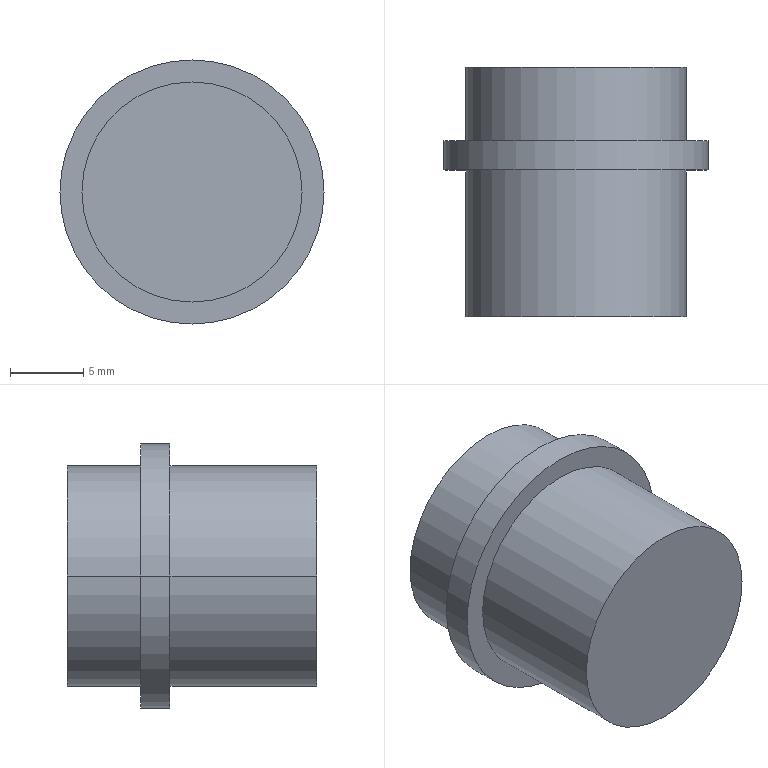Component | SolidWorks | AviationPlug-1 | 1 solid | 24 faces | box 18 x 17 x 18 mm | volume 1920 mm3 | cylinder 15 | plane 9 | commonest cylinder face diameters 2 x7 15 x4 13 x2 18 x2
build123d program:
from build123d import *

# Parameters (mm, degrees)
SKETCH1_R           = 9
BOSS_EXTRUDE1_DEPTH = 2
SKETCH2_R           = 7.5
BOSS_EXTRUDE2_DEPTH = 5
BOSS_EXTRUDE3_START = 10
SKETCH4_R           = 7.5
BOSS_EXTRUDE3_DEPTH = 10
SKETCH3_R           = 1
CUT_EXTRUDE1_DEPTH  = 10
SKETCH5_R           = 6.5
CUT_EXTRUDE2_DEPTH  = 2


with BuildPart() as part:
    # Sketch1 → Boss-Extrude1 (new body)
    with BuildSketch(Plane.XY):
        Circle(SKETCH1_R)
    extrude(amount=BOSS_EXTRUDE1_DEPTH)

    # Sketch2 → Boss-Extrude2 (add)
    with BuildSketch(Plane.XY.offset(2)):
        Circle(SKETCH2_R)
    extrude(amount=BOSS_EXTRUDE2_DEPTH)

    # Sketch4 → Boss-Extrude3 (add)
    with BuildSketch(Plane(origin=(0, 0, 0), x_dir=(-1, 0, 0), z_dir=(0, 0, -1)).offset(BOSS_EXTRUDE3_START)):
        with Locations(Location((0, 0, 0), (0, 0, 180))):
            Circle(SKETCH4_R)
    extrude(amount=-BOSS_EXTRUDE3_DEPTH)

    # Sketch3 → Cut-Extrude1 (cut)
    with BuildSketch(Plane.XY.offset(7)):
        with BuildLine():
            ThreePointArc((-0.997, 6.423), (0, -6.5), (0.997, 6.423))
            ThreePointArc((0.997, 6.423), (0, 5.5), (-0.997, 6.423))
        make_face()
        with Locations((-3.25, 1.876)):
            Circle(SKETCH3_R, mode=Mode.SUBTRACT)
        with Locations((3.25, 1.876)):
            Circle(SKETCH3_R, mode=Mode.SUBTRACT)
        with Locations((0, -3.753)):
            Circle(SKETCH3_R, mode=Mode.SUBTRACT)
    extrude(amount=-CUT_EXTRUDE1_DEPTH, mode=Mode.SUBTRACT)

    # Sketch5 → Cut-Extrude2 (cut)
    with BuildSketch(Plane.XY.offset(7)):
        Circle(SKETCH5_R)
    extrude(amount=-CUT_EXTRUDE2_DEPTH, mode=Mode.SUBTRACT)


solid = part.part

# Placed as in the assembly
solid = solid.moved(Location((1197.686, 1563.312, 2265.983), (-90, 0, 0)))
STEP:
#1=CARTESIAN_POINT('',(46.897,61.43,89.212));
#2=VERTEX_POINT('',#1);
#3=CARTESIAN_POINT('',(47.409,61.43,89.212));
#4=VERTEX_POINT('',#3);
#5=CARTESIAN_POINT('',(47.153,61.43,89.212));
#6=DIRECTION('',(0.,1.,0.));
#7=DIRECTION('',(1.,0.,0.));
#8=AXIS2_PLACEMENT_3D('',#5,#6,#7);
#9=CIRCLE('',#8,0.2559);
#10=EDGE_CURVE('',#2,#4,#9,.T.);
#11=ORIENTED_EDGE('',*,*,#10,.F.);
#12=CARTESIAN_POINT('',(46.897,61.823,89.212));
#13=VERTEX_POINT('',#12);
#14=CARTESIAN_POINT('',(46.897,61.43,89.212));
#15=DIRECTION('',(0.,1.,0.));
#16=VECTOR('',#15,39.37);
#17=LINE('',#14,#16);
#18=EDGE_CURVE('',#2,#13,#17,.T.);
#19=ORIENTED_EDGE('',*,*,#18,.T.);
#20=CARTESIAN_POINT('',(47.409,61.823,89.212));
#21=VERTEX_POINT('',#20);
#22=CARTESIAN_POINT('',(47.153,61.823,89.212));
#23=DIRECTION('',(0.,1.,0.));
#24=DIRECTION('',(1.,0.,0.));
#25=AXIS2_PLACEMENT_3D('',#22,#23,#24);
#26=CIRCLE('',#25,0.2559);
#27=EDGE_CURVE('',#13,#21,#26,.T.);
#28=ORIENTED_EDGE('',*,*,#27,.T.);
#29=CARTESIAN_POINT('',(47.409,61.43,89.212));
#30=DIRECTION('',(0.,1.,0.));
#31=VECTOR('',#30,39.37);
#32=LINE('',#29,#31);
#33=EDGE_CURVE('',#4,#21,#32,.T.);
#34=ORIENTED_EDGE('',*,*,#33,.F.);
#35=EDGE_LOOP('',(#11,#19,#28,#34));
#36=FACE_OUTER_BOUND('',#35,.T.);
#37=CARTESIAN_POINT('',(47.153,61.43,89.212));
#38=DIRECTION('',(0.,1.,0.));
#39=DIRECTION('',(1.,0.,0.));
#40=AXIS2_PLACEMENT_3D('',#37,#38,#39);
#41=CYLINDRICAL_SURFACE('',#40,0.2559);
#42=ADVANCED_FACE('',(#36),#41,.F.);
#43=CARTESIAN_POINT('',(46.858,61.154,89.212));
#44=VERTEX_POINT('',#43);
#45=CARTESIAN_POINT('',(47.448,61.154,89.212));
#46=VERTEX_POINT('',#45);
#47=CARTESIAN_POINT('',(47.153,61.154,89.212));
#48=DIRECTION('',(0.,-1.,-0.));
#49=DIRECTION('',(-1.,0.,0.));
#50=AXIS2_PLACEMENT_3D('',#47,#48,#49);
#51=CIRCLE('',#50,0.2953);
#52=EDGE_CURVE('',#44,#46,#51,.T.);
#53=ORIENTED_EDGE('',*,*,#52,.F.);
#54=CARTESIAN_POINT('',(46.858,61.548,89.212));
#55=VERTEX_POINT('',#54);
#56=CARTESIAN_POINT('',(46.858,61.154,89.212));
#57=DIRECTION('',(0.,1.,0.));
#58=VECTOR('',#57,39.37);
#59=LINE('',#56,#58);
#60=EDGE_CURVE('',#44,#55,#59,.T.);
#61=ORIENTED_EDGE('',*,*,#60,.T.);
#62=CARTESIAN_POINT('',(47.448,61.548,89.212));
#63=VERTEX_POINT('',#62);
#64=CARTESIAN_POINT('',(47.153,61.548,89.212));
#65=DIRECTION('',(0.,-1.,-0.));
#66=DIRECTION('',(1.,0.,0.));
#67=AXIS2_PLACEMENT_3D('',#64,#65,#66);
#68=CIRCLE('',#67,0.2953);
#69=EDGE_CURVE('',#55,#63,#68,.T.);
#70=ORIENTED_EDGE('',*,*,#69,.T.);
#71=CARTESIAN_POINT('',(47.448,61.154,89.212));
#72=DIRECTION('',(0.,1.,0.));
#73=VECTOR('',#72,39.37);
#74=LINE('',#71,#73);
#75=EDGE_CURVE('',#46,#63,#74,.T.);
#76=ORIENTED_EDGE('',*,*,#75,.F.);
#77=EDGE_LOOP('',(#53,#61,#70,#76));
#78=FACE_OUTER_BOUND('',#77,.T.);
#79=CARTESIAN_POINT('',(47.153,61.154,89.212));
#80=DIRECTION('',(0.,1.,0.));
#81=DIRECTION('',(1.,0.,0.));
#82=AXIS2_PLACEMENT_3D('',#79,#80,#81);
#83=CYLINDRICAL_SURFACE('',#82,0.2953);
#84=ADVANCED_FACE('',(#78),#83,.T.);
#85=CARTESIAN_POINT('',(47.448,61.823,89.212));
#86=VERTEX_POINT('',#85);
#87=CARTESIAN_POINT('',(46.858,61.823,89.212));
#88=VERTEX_POINT('',#87);
#89=CARTESIAN_POINT('',(47.153,61.823,89.212));
#90=DIRECTION('',(0.,1.,0.));
#91=DIRECTION('',(1.,0.,0.));
#92=AXIS2_PLACEMENT_3D('',#89,#90,#91);
#93=CIRCLE('',#92,0.2953);
#94=EDGE_CURVE('',#86,#88,#93,.T.);
#95=ORIENTED_EDGE('',*,*,#94,.F.);
#96=CARTESIAN_POINT('',(47.448,61.626,89.212));
#97=VERTEX_POINT('',#96);
#98=CARTESIAN_POINT('',(47.448,61.823,89.212));
#99=DIRECTION('',(0.,-1.,-0.));
#100=VECTOR('',#99,39.37);
#101=LINE('',#98,#100);
#102=EDGE_CURVE('',#86,#97,#101,.T.);
#103=ORIENTED_EDGE('',*,*,#102,.T.);
#104=CARTESIAN_POINT('',(46.858,61.626,89.212));
#105=VERTEX_POINT('',#104);
#106=CARTESIAN_POINT('',(47.153,61.626,89.212));
#107=DIRECTION('',(0.,1.,0.));
#108=DIRECTION('',(1.,0.,0.));
#109=AXIS2_PLACEMENT_3D('',#106,#107,#108);
#110=CIRCLE('',#109,0.2953);
#111=EDGE_CURVE('',#97,#105,#110,.T.);
#112=ORIENTED_EDGE('',*,*,#111,.T.);
#113=CARTESIAN_POINT('',(46.858,61.823,89.212));
#114=DIRECTION('',(0.,-1.,-0.));
#115=VECTOR('',#114,39.37);
#116=LINE('',#113,#115);
#117=EDGE_CURVE('',#88,#105,#116,.T.);
#118=ORIENTED_EDGE('',*,*,#117,.F.);
#119=EDGE_LOOP('',(#95,#103,#112,#118));
#120=FACE_OUTER_BOUND('',#119,.T.);
#121=CARTESIAN_POINT('',(47.153,61.823,89.212));
#122=DIRECTION('',(0.,-1.,-0.));
#123=DIRECTION('',(-1.,0.,0.));
#124=AXIS2_PLACEMENT_3D('',#121,#122,#123);
#125=CYLINDRICAL_SURFACE('',#124,0.2953);
#126=ADVANCED_FACE('',(#120),#125,.T.);
#127=CARTESIAN_POINT('',(47.507,61.626,89.212));
#128=VERTEX_POINT('',#127);
#129=CARTESIAN_POINT('',(46.799,61.626,89.212));
#130=VERTEX_POINT('',#129);
#131=CARTESIAN_POINT('',(47.153,61.626,89.212));
#132=DIRECTION('',(0.,1.,0.));
#133=DIRECTION('',(1.,0.,0.));
#134=AXIS2_PLACEMENT_3D('',#131,#132,#133);
#135=CIRCLE('',#134,0.3543);
#136=EDGE_CURVE('',#128,#130,#135,.T.);
#137=ORIENTED_EDGE('',*,*,#136,.F.);
#138=CARTESIAN_POINT('',(47.507,61.548,89.212));
#139=VERTEX_POINT('',#138);
#140=CARTESIAN_POINT('',(47.507,61.626,89.212));
#141=DIRECTION('',(0.,-1.,-0.));
#142=VECTOR('',#141,39.37);
#143=LINE('',#140,#142);
#144=EDGE_CURVE('',#128,#139,#143,.T.);
#145=ORIENTED_EDGE('',*,*,#144,.T.);
#146=CARTESIAN_POINT('',(46.799,61.548,89.212));
#147=VERTEX_POINT('',#146);
#148=CARTESIAN_POINT('',(47.153,61.548,89.212));
#149=DIRECTION('',(0.,1.,0.));
#150=DIRECTION('',(1.,0.,0.));
#151=AXIS2_PLACEMENT_3D('',#148,#149,#150);
#152=CIRCLE('',#151,0.3543);
#153=EDGE_CURVE('',#139,#147,#152,.T.);
#154=ORIENTED_EDGE('',*,*,#153,.T.);
#155=CARTESIAN_POINT('',(46.799,61.626,89.212));
#156=DIRECTION('',(0.,-1.,-0.));
#157=VECTOR('',#156,39.37);
#158=LINE('',#155,#157);
#159=EDGE_CURVE('',#130,#147,#158,.T.);
#160=ORIENTED_EDGE('',*,*,#159,.F.);
#161=EDGE_LOOP('',(#137,#145,#154,#160));
#162=FACE_OUTER_BOUND('',#161,.T.);
#163=CARTESIAN_POINT('',(47.153,61.626,89.212));
#164=DIRECTION('',(0.,-1.,-0.));
#165=DIRECTION('',(-1.,0.,0.));
#166=AXIS2_PLACEMENT_3D('',#163,#164,#165);
#167=CYLINDRICAL_SURFACE('',#166,0.3543);
#168=ADVANCED_FACE('',(#162),#167,.T.);
#169=CARTESIAN_POINT('',(47.192,61.43,89.36));
#170=VERTEX_POINT('',#169);
#171=CARTESIAN_POINT('',(47.114,61.43,89.36));
#172=VERTEX_POINT('',#171);
#173=CARTESIAN_POINT('',(47.153,61.43,89.36));
#174=DIRECTION('',(0.,1.,0.));
#175=DIRECTION('',(1.,0.,0.));
#176=AXIS2_PLACEMENT_3D('',#173,#174,#175);
#177=CIRCLE('',#176,0.03937);
#178=EDGE_CURVE('',#170,#172,#177,.T.);
#179=ORIENTED_EDGE('',*,*,#178,.T.);
#180=CARTESIAN_POINT('',(47.114,61.745,89.36));
#181=VERTEX_POINT('',#180);
#182=CARTESIAN_POINT('',(47.114,61.43,89.36));
#183=DIRECTION('',(0.,1.,0.));
#184=VECTOR('',#183,39.37);
#185=LINE('',#182,#184);
#186=EDGE_CURVE('',#172,#181,#185,.T.);
#187=ORIENTED_EDGE('',*,*,#186,.T.);
#188=CARTESIAN_POINT('',(47.192,61.745,89.36));
#189=VERTEX_POINT('',#188);
#190=CARTESIAN_POINT('',(47.153,61.745,89.36));
#191=DIRECTION('',(0.,-1.,-0.));
#192=DIRECTION('',(1.,0.,0.));
#193=AXIS2_PLACEMENT_3D('',#190,#191,#192);
#194=CIRCLE('',#193,0.03937);
#195=EDGE_CURVE('',#181,#189,#194,.T.);
#196=ORIENTED_EDGE('',*,*,#195,.T.);
#197=CARTESIAN_POINT('',(47.192,61.43,89.36));
#198=DIRECTION('',(0.,1.,0.));
#199=VECTOR('',#198,39.37);
#200=LINE('',#197,#199);
#201=EDGE_CURVE('',#170,#189,#200,.T.);
#202=ORIENTED_EDGE('',*,*,#201,.F.);
#203=EDGE_LOOP('',(#179,#187,#196,#202));
#204=FACE_OUTER_BOUND('',#203,.T.);
#205=CARTESIAN_POINT('',(47.153,61.43,89.36));
#206=DIRECTION('',(0.,1.,0.));
#207=DIRECTION('',(1.,0.,0.));
#208=AXIS2_PLACEMENT_3D('',#205,#206,#207);
#209=CYLINDRICAL_SURFACE('',#208,0.03937);
#210=ADVANCED_FACE('',(#204),#209,.T.);
#211=CARTESIAN_POINT('',(47.32,61.43,89.138));
#212=VERTEX_POINT('',#211);
#213=CARTESIAN_POINT('',(47.242,61.43,89.138));
#214=VERTEX_POINT('',#213);
#215=CARTESIAN_POINT('',(47.281,61.43,89.138));
#216=DIRECTION('',(0.,1.,0.));
#217=DIRECTION('',(1.,0.,0.));
#218=AXIS2_PLACEMENT_3D('',#215,#216,#217);
#219=CIRCLE('',#218,0.03937);
#220=EDGE_CURVE('',#212,#214,#219,.T.);
#221=ORIENTED_EDGE('',*,*,#220,.T.);
#222=CARTESIAN_POINT('',(47.242,61.745,89.138));
#223=VERTEX_POINT('',#222);
#224=CARTESIAN_POINT('',(47.242,61.43,89.138));
#225=DIRECTION('',(0.,1.,0.));
#226=VECTOR('',#225,39.37);
#227=LINE('',#224,#226);
#228=EDGE_CURVE('',#214,#223,#227,.T.);
#229=ORIENTED_EDGE('',*,*,#228,.T.);
#230=CARTESIAN_POINT('',(47.32,61.745,89.138));
#231=VERTEX_POINT('',#230);
#232=CARTESIAN_POINT('',(47.281,61.745,89.138));
#233=DIRECTION('',(0.,-1.,-0.));
#234=DIRECTION('',(1.,0.,0.));
#235=AXIS2_PLACEMENT_3D('',#232,#233,#234);
#236=CIRCLE('',#235,0.03937);
#237=EDGE_CURVE('',#223,#231,#236,.T.);
#238=ORIENTED_EDGE('',*,*,#237,.T.);
#239=CARTESIAN_POINT('',(47.32,61.43,89.138));
#240=DIRECTION('',(0.,1.,0.));
#241=VECTOR('',#240,39.37);
#242=LINE('',#239,#241);
#243=EDGE_CURVE('',#212,#231,#242,.T.);
#244=ORIENTED_EDGE('',*,*,#243,.F.);
#245=EDGE_LOOP('',(#221,#229,#238,#244));
#246=FACE_OUTER_BOUND('',#245,.T.);
#247=CARTESIAN_POINT('',(47.281,61.43,89.138));
#248=DIRECTION('',(0.,1.,0.));
#249=DIRECTION('',(1.,0.,0.));
#250=AXIS2_PLACEMENT_3D('',#247,#248,#249);
#251=CYLINDRICAL_SURFACE('',#250,0.03937);
#252=ADVANCED_FACE('',(#246),#251,.T.);
#253=CARTESIAN_POINT('',(47.064,61.43,89.138));
#254=VERTEX_POINT('',#253);
#255=CARTESIAN_POINT('',(46.986,61.43,89.138));
#256=VERTEX_POINT('',#255);
#257=CARTESIAN_POINT('',(47.025,61.43,89.138));
#258=DIRECTION('',(0.,1.,0.));
#259=DIRECTION('',(1.,0.,0.));
#260=AXIS2_PLACEMENT_3D('',#257,#258,#259);
#261=CIRCLE('',#260,0.03937);
#262=EDGE_CURVE('',#254,#256,#261,.T.);
#263=ORIENTED_EDGE('',*,*,#262,.T.);
#264=CARTESIAN_POINT('',(46.986,61.745,89.138));
#265=VERTEX_POINT('',#264);
#266=CARTESIAN_POINT('',(46.986,61.43,89.138));
#267=DIRECTION('',(0.,1.,0.));
#268=VECTOR('',#267,39.37);
#269=LINE('',#266,#268);
#270=EDGE_CURVE('',#256,#265,#269,.T.);
#271=ORIENTED_EDGE('',*,*,#270,.T.);
#272=CARTESIAN_POINT('',(47.064,61.745,89.138));
#273=VERTEX_POINT('',#272);
#274=CARTESIAN_POINT('',(47.025,61.745,89.138));
#275=DIRECTION('',(0.,-1.,-0.));
#276=DIRECTION('',(1.,0.,0.));
#277=AXIS2_PLACEMENT_3D('',#274,#275,#276);
#278=CIRCLE('',#277,0.03937);
#279=EDGE_CURVE('',#265,#273,#278,.T.);
#280=ORIENTED_EDGE('',*,*,#279,.T.);
#281=CARTESIAN_POINT('',(47.064,61.43,89.138));
#282=DIRECTION('',(0.,1.,0.));
#283=VECTOR('',#282,39.37);
#284=LINE('',#281,#283);
#285=EDGE_CURVE('',#254,#273,#284,.T.);
#286=ORIENTED_EDGE('',*,*,#285,.F.);
#287=EDGE_LOOP('',(#263,#271,#280,#286));
#288=FACE_OUTER_BOUND('',#287,.T.);
#289=CARTESIAN_POINT('',(47.025,61.43,89.138));
#290=DIRECTION('',(0.,1.,0.));
#291=DIRECTION('',(1.,0.,0.));
#292=AXIS2_PLACEMENT_3D('',#289,#290,#291);
#293=CYLINDRICAL_SURFACE('',#292,0.03937);
#294=ADVANCED_FACE('',(#288),#293,.T.);
#295=CARTESIAN_POINT('',(47.114,61.745,88.959));
#296=VERTEX_POINT('',#295);
#297=CARTESIAN_POINT('',(47.192,61.745,88.959));
#298=VERTEX_POINT('',#297);
#299=CARTESIAN_POINT('',(47.153,61.745,88.956));
#300=DIRECTION('',(0.,1.,0.));
#301=DIRECTION('',(1.,0.,0.));
#302=AXIS2_PLACEMENT_3D('',#299,#300,#301);
#303=CIRCLE('',#302,0.03937);
#304=EDGE_CURVE('',#296,#298,#303,.T.);
#305=ORIENTED_EDGE('',*,*,#304,.F.);
#306=CARTESIAN_POINT('',(47.114,61.43,88.959));
#307=VERTEX_POINT('',#306);
#308=CARTESIAN_POINT('',(47.114,61.43,88.959));
#309=DIRECTION('',(0.,1.,0.));
#310=VECTOR('',#309,39.37);
#311=LINE('',#308,#310);
#312=EDGE_CURVE('',#307,#296,#311,.T.);
#313=ORIENTED_EDGE('',*,*,#312,.F.);
#314=CARTESIAN_POINT('',(47.192,61.43,88.959));
#315=VERTEX_POINT('',#314);
#316=CARTESIAN_POINT('',(47.153,61.43,88.956));
#317=DIRECTION('',(0.,-1.,-0.));
#318=DIRECTION('',(1.,0.,0.));
#319=AXIS2_PLACEMENT_3D('',#316,#317,#318);
#320=CIRCLE('',#319,0.03937);
#321=EDGE_CURVE('',#315,#307,#320,.T.);
#322=ORIENTED_EDGE('',*,*,#321,.F.);
#323=CARTESIAN_POINT('',(47.192,61.43,88.959));
#324=DIRECTION('',(0.,1.,0.));
#325=VECTOR('',#324,39.37);
#326=LINE('',#323,#325);
#327=EDGE_CURVE('',#315,#298,#326,.T.);
#328=ORIENTED_EDGE('',*,*,#327,.T.);
#329=EDGE_LOOP('',(#305,#313,#322,#328));
#330=FACE_OUTER_BOUND('',#329,.T.);
#331=CARTESIAN_POINT('',(47.153,61.43,88.956));
#332=DIRECTION('',(0.,1.,0.));
#333=DIRECTION('',(1.,0.,0.));
#334=AXIS2_PLACEMENT_3D('',#331,#332,#333);
#335=CYLINDRICAL_SURFACE('',#334,0.03937);
#336=ADVANCED_FACE('',(#330),#335,.T.);
#337=ORIENTED_EDGE('',*,*,#270,.F.);
#338=CARTESIAN_POINT('',(47.025,61.43,89.138));
#339=DIRECTION('',(0.,1.,0.));
#340=DIRECTION('',(1.,0.,0.));
#341=AXIS2_PLACEMENT_3D('',#338,#339,#340);
#342=CIRCLE('',#341,0.03937);
#343=EDGE_CURVE('',#256,#254,#342,.T.);
#344=ORIENTED_EDGE('',*,*,#343,.T.);
#345=ORIENTED_EDGE('',*,*,#285,.T.);
#346=CARTESIAN_POINT('',(47.025,61.745,89.138));
#347=DIRECTION('',(0.,-1.,-0.));
#348=DIRECTION('',(1.,0.,0.));
#349=AXIS2_PLACEMENT_3D('',#346,#347,#348);
#350=CIRCLE('',#349,0.03937);
#351=EDGE_CURVE('',#273,#265,#350,.T.);
#352=ORIENTED_EDGE('',*,*,#351,.T.);
#353=EDGE_LOOP('',(#337,#344,#345,#352));
#354=FACE_OUTER_BOUND('',#353,.T.);
#355=CARTESIAN_POINT('',(47.025,61.43,89.138));
#356=DIRECTION('',(0.,1.,0.));
#357=DIRECTION('',(1.,0.,0.));
#358=AXIS2_PLACEMENT_3D('',#355,#356,#357);
#359=CYLINDRICAL_SURFACE('',#358,0.03937);
#360=ADVANCED_FACE('',(#354),#359,.T.);
#361=ORIENTED_EDGE('',*,*,#228,.F.);
#362=CARTESIAN_POINT('',(47.281,61.43,89.138));
#363=DIRECTION('',(0.,1.,0.));
#364=DIRECTION('',(1.,0.,0.));
#365=AXIS2_PLACEMENT_3D('',#362,#363,#364);
#366=CIRCLE('',#365,0.03937);
#367=EDGE_CURVE('',#214,#212,#366,.T.);
#368=ORIENTED_EDGE('',*,*,#367,.T.);
#369=ORIENTED_EDGE('',*,*,#243,.T.);
#370=CARTESIAN_POINT('',(47.281,61.745,89.138));
#371=DIRECTION('',(0.,-1.,-0.));
#372=DIRECTION('',(1.,0.,0.));
#373=AXIS2_PLACEMENT_3D('',#370,#371,#372);
#374=CIRCLE('',#373,0.03937);
#375=EDGE_CURVE('',#231,#223,#374,.T.);
#376=ORIENTED_EDGE('',*,*,#375,.T.);
#377=EDGE_LOOP('',(#361,#368,#369,#376));
#378=FACE_OUTER_BOUND('',#377,.T.);
#379=CARTESIAN_POINT('',(47.281,61.43,89.138));
#380=DIRECTION('',(0.,1.,0.));
#381=DIRECTION('',(1.,0.,0.));
#382=AXIS2_PLACEMENT_3D('',#379,#380,#381);
#383=CYLINDRICAL_SURFACE('',#382,0.03937);
#384=ADVANCED_FACE('',(#378),#383,.T.);
#385=ORIENTED_EDGE('',*,*,#186,.F.);
#386=CARTESIAN_POINT('',(47.153,61.43,89.36));
#387=DIRECTION('',(0.,1.,0.));
#388=DIRECTION('',(1.,0.,0.));
#389=AXIS2_PLACEMENT_3D('',#386,#387,#388);
#390=CIRCLE('',#389,0.03937);
#391=EDGE_CURVE('',#172,#170,#390,.T.);
#392=ORIENTED_EDGE('',*,*,#391,.T.);
#393=ORIENTED_EDGE('',*,*,#201,.T.);
#394=CARTESIAN_POINT('',(47.153,61.745,89.36));
#395=DIRECTION('',(0.,-1.,-0.));
#396=DIRECTION('',(1.,0.,0.));
#397=AXIS2_PLACEMENT_3D('',#394,#395,#396);
#398=CIRCLE('',#397,0.03937);
#399=EDGE_CURVE('',#189,#181,#398,.T.);
#400=ORIENTED_EDGE('',*,*,#399,.T.);
#401=EDGE_LOOP('',(#385,#392,#393,#400));
#402=FACE_OUTER_BOUND('',#401,.T.);
#403=CARTESIAN_POINT('',(47.153,61.43,89.36));
#404=DIRECTION('',(0.,1.,0.));
#405=DIRECTION('',(1.,0.,0.));
#406=AXIS2_PLACEMENT_3D('',#403,#404,#405);
#407=CYLINDRICAL_SURFACE('',#406,0.03937);
#408=ADVANCED_FACE('',(#402),#407,.T.);
#409=ORIENTED_EDGE('',*,*,#144,.F.);
#410=CARTESIAN_POINT('',(47.153,61.626,89.212));
#411=DIRECTION('',(0.,1.,0.));
#412=DIRECTION('',(1.,0.,0.));
#413=AXIS2_PLACEMENT_3D('',#410,#411,#412);
#414=CIRCLE('',#413,0.3543);
#415=EDGE_CURVE('',#130,#128,#414,.T.);
#416=ORIENTED_EDGE('',*,*,#415,.F.);
#417=ORIENTED_EDGE('',*,*,#159,.T.);
#418=CARTESIAN_POINT('',(47.153,61.548,89.212));
#419=DIRECTION('',(0.,1.,0.));
#420=DIRECTION('',(1.,0.,0.));
#421=AXIS2_PLACEMENT_3D('',#418,#419,#420);
#422=CIRCLE('',#421,0.3543);
#423=EDGE_CURVE('',#147,#139,#422,.T.);
#424=ORIENTED_EDGE('',*,*,#423,.T.);
#425=EDGE_LOOP('',(#409,#416,#417,#424));
#426=FACE_OUTER_BOUND('',#425,.T.);
#427=CARTESIAN_POINT('',(47.153,61.626,89.212));
#428=DIRECTION('',(0.,-1.,-0.));
#429=DIRECTION('',(-1.,0.,0.));
#430=AXIS2_PLACEMENT_3D('',#427,#428,#429);
#431=CYLINDRICAL_SURFACE('',#430,0.3543);
#432=ADVANCED_FACE('',(#426),#431,.T.);
#433=CARTESIAN_POINT('',(47.153,61.626,89.212));
#434=DIRECTION('',(0.,1.,0.));
#435=DIRECTION('',(1.,0.,0.));
#436=AXIS2_PLACEMENT_3D('',#433,#434,#435);
#437=CIRCLE('',#436,0.2953);
#438=EDGE_CURVE('',#105,#97,#437,.T.);
#439=ORIENTED_EDGE('',*,*,#438,.F.);
#440=ORIENTED_EDGE('',*,*,#111,.F.);
#441=EDGE_LOOP('',(#439,#440));
#442=FACE_BOUND('',#441,.T.);
#443=ORIENTED_EDGE('',*,*,#415,.T.);
#444=ORIENTED_EDGE('',*,*,#136,.T.);
#445=EDGE_LOOP('',(#443,#444));
#446=FACE_OUTER_BOUND('',#445,.T.);
#447=CARTESIAN_POINT('',(47.153,61.626,89.212));
#448=DIRECTION('',(0.,1.,0.));
#449=DIRECTION('',(1.,0.,0.));
#450=AXIS2_PLACEMENT_3D('',#447,#448,#449);
#451=PLANE('',#450);
#452=ADVANCED_FACE('',(#442,#446),#451,.T.);
#453=CARTESIAN_POINT('',(47.153,61.548,89.212));
#454=DIRECTION('',(0.,-1.,-0.));
#455=DIRECTION('',(1.,0.,0.));
#456=AXIS2_PLACEMENT_3D('',#453,#454,#455);
#457=CIRCLE('',#456,0.2953);
#458=EDGE_CURVE('',#63,#55,#457,.T.);
#459=ORIENTED_EDGE('',*,*,#458,.F.);
#460=ORIENTED_EDGE('',*,*,#69,.F.);
#461=EDGE_LOOP('',(#459,#460));
#462=FACE_BOUND('',#461,.T.);
#463=ORIENTED_EDGE('',*,*,#423,.F.);
#464=ORIENTED_EDGE('',*,*,#153,.F.);
#465=EDGE_LOOP('',(#463,#464));
#466=FACE_OUTER_BOUND('',#465,.T.);
#467=CARTESIAN_POINT('',(47.153,61.548,89.212));
#468=DIRECTION('',(0.,1.,0.));
#469=DIRECTION('',(1.,0.,0.));
#470=AXIS2_PLACEMENT_3D('',#467,#468,#469);
#471=PLANE('',#470);
#472=ADVANCED_FACE('',(#462,#466),#471,.F.);
#473=ORIENTED_EDGE('',*,*,#102,.F.);
#474=CARTESIAN_POINT('',(47.153,61.823,89.212));
#475=DIRECTION('',(0.,1.,0.));
#476=DIRECTION('',(1.,0.,0.));
#477=AXIS2_PLACEMENT_3D('',#474,#475,#476);
#478=CIRCLE('',#477,0.2953);
#479=EDGE_CURVE('',#88,#86,#478,.T.);
#480=ORIENTED_EDGE('',*,*,#479,.F.);
#481=ORIENTED_EDGE('',*,*,#117,.T.);
#482=ORIENTED_EDGE('',*,*,#438,.T.);
#483=EDGE_LOOP('',(#473,#480,#481,#482));
#484=FACE_OUTER_BOUND('',#483,.T.);
#485=CARTESIAN_POINT('',(47.153,61.823,89.212));
#486=DIRECTION('',(0.,-1.,-0.));
#487=DIRECTION('',(-1.,0.,0.));
#488=AXIS2_PLACEMENT_3D('',#485,#486,#487);
#489=CYLINDRICAL_SURFACE('',#488,0.2953);
#490=ADVANCED_FACE('',(#484),#489,.T.);
#491=CARTESIAN_POINT('',(47.153,61.823,89.212));
#492=DIRECTION('',(0.,1.,0.));
#493=DIRECTION('',(1.,0.,0.));
#494=AXIS2_PLACEMENT_3D('',#491,#492,#493);
#495=CIRCLE('',#494,0.2559);
#496=EDGE_CURVE('',#21,#13,#495,.T.);
#497=ORIENTED_EDGE('',*,*,#496,.F.);
#498=ORIENTED_EDGE('',*,*,#27,.F.);
#499=EDGE_LOOP('',(#497,#498));
#500=FACE_BOUND('',#499,.T.);
#501=ORIENTED_EDGE('',*,*,#479,.T.);
#502=ORIENTED_EDGE('',*,*,#94,.T.);
#503=EDGE_LOOP('',(#501,#502));
#504=FACE_OUTER_BOUND('',#503,.T.);
#505=CARTESIAN_POINT('',(47.153,61.823,89.212));
#506=DIRECTION('',(0.,1.,0.));
#507=DIRECTION('',(1.,0.,0.));
#508=AXIS2_PLACEMENT_3D('',#505,#506,#507);
#509=PLANE('',#508);
#510=ADVANCED_FACE('',(#500,#504),#509,.T.);
#511=ORIENTED_EDGE('',*,*,#60,.F.);
#512=CARTESIAN_POINT('',(47.153,61.154,89.212));
#513=DIRECTION('',(0.,-1.,-0.));
#514=DIRECTION('',(-1.,0.,0.));
#515=AXIS2_PLACEMENT_3D('',#512,#513,#514);
#516=CIRCLE('',#515,0.2953);
#517=EDGE_CURVE('',#46,#44,#516,.T.);
#518=ORIENTED_EDGE('',*,*,#517,.F.);
#519=ORIENTED_EDGE('',*,*,#75,.T.);
#520=ORIENTED_EDGE('',*,*,#458,.T.);
#521=EDGE_LOOP('',(#511,#518,#519,#520));
#522=FACE_OUTER_BOUND('',#521,.T.);
#523=CARTESIAN_POINT('',(47.153,61.154,89.212));
#524=DIRECTION('',(0.,1.,0.));
#525=DIRECTION('',(1.,0.,0.));
#526=AXIS2_PLACEMENT_3D('',#523,#524,#525);
#527=CYLINDRICAL_SURFACE('',#526,0.2953);
#528=ADVANCED_FACE('',(#522),#527,.T.);
#529=ORIENTED_EDGE('',*,*,#517,.T.);
#530=ORIENTED_EDGE('',*,*,#52,.T.);
#531=EDGE_LOOP('',(#529,#530));
#532=FACE_OUTER_BOUND('',#531,.T.);
#533=CARTESIAN_POINT('',(47.153,61.154,89.212));
#534=DIRECTION('',(0.,-1.,-0.));
#535=DIRECTION('',(-1.,0.,0.));
#536=AXIS2_PLACEMENT_3D('',#533,#534,#535);
#537=PLANE('',#536);
#538=ADVANCED_FACE('',(#532),#537,.T.);
#539=ORIENTED_EDGE('',*,*,#18,.F.);
#540=CARTESIAN_POINT('',(47.153,61.43,89.212));
#541=DIRECTION('',(0.,1.,0.));
#542=DIRECTION('',(1.,0.,0.));
#543=AXIS2_PLACEMENT_3D('',#540,#541,#542);
#544=CIRCLE('',#543,0.2559);
#545=EDGE_CURVE('',#307,#2,#544,.T.);
#546=ORIENTED_EDGE('',*,*,#545,.F.);
#547=ORIENTED_EDGE('',*,*,#312,.T.);
#548=CARTESIAN_POINT('',(47.153,61.745,89.212));
#549=DIRECTION('',(0.,1.,0.));
#550=DIRECTION('',(1.,0.,0.));
#551=AXIS2_PLACEMENT_3D('',#548,#549,#550);
#552=CIRCLE('',#551,0.2559);
#553=EDGE_CURVE('',#298,#296,#552,.T.);
#554=ORIENTED_EDGE('',*,*,#553,.F.);
#555=ORIENTED_EDGE('',*,*,#327,.F.);
#556=CARTESIAN_POINT('',(47.153,61.43,89.212));
#557=DIRECTION('',(0.,1.,0.));
#558=DIRECTION('',(1.,0.,0.));
#559=AXIS2_PLACEMENT_3D('',#556,#557,#558);
#560=CIRCLE('',#559,0.2559);
#561=EDGE_CURVE('',#4,#315,#560,.T.);
#562=ORIENTED_EDGE('',*,*,#561,.F.);
#563=ORIENTED_EDGE('',*,*,#33,.T.);
#564=ORIENTED_EDGE('',*,*,#496,.T.);
#565=EDGE_LOOP('',(#539,#546,#547,#554,#555,#562,#563,#564));
#566=FACE_OUTER_BOUND('',#565,.T.);
#567=CARTESIAN_POINT('',(47.153,61.43,89.212));
#568=DIRECTION('',(0.,1.,0.));
#569=DIRECTION('',(1.,0.,0.));
#570=AXIS2_PLACEMENT_3D('',#567,#568,#569);
#571=CYLINDRICAL_SURFACE('',#570,0.2559);
#572=ADVANCED_FACE('',(#566),#571,.F.);
#573=ORIENTED_EDGE('',*,*,#178,.F.);
#574=ORIENTED_EDGE('',*,*,#391,.F.);
#575=EDGE_LOOP('',(#573,#574));
#576=FACE_BOUND('',#575,.T.);
#577=ORIENTED_EDGE('',*,*,#220,.F.);
#578=ORIENTED_EDGE('',*,*,#367,.F.);
#579=EDGE_LOOP('',(#577,#578));
#580=FACE_BOUND('',#579,.T.);
#581=ORIENTED_EDGE('',*,*,#262,.F.);
#582=ORIENTED_EDGE('',*,*,#343,.F.);
#583=EDGE_LOOP('',(#581,#582));
#584=FACE_BOUND('',#583,.T.);
#585=ORIENTED_EDGE('',*,*,#321,.T.);
#586=ORIENTED_EDGE('',*,*,#545,.T.);
#587=ORIENTED_EDGE('',*,*,#10,.T.);
#588=ORIENTED_EDGE('',*,*,#561,.T.);
#589=EDGE_LOOP('',(#585,#586,#587,#588));
#590=FACE_OUTER_BOUND('',#589,.T.);
#591=CARTESIAN_POINT('',(47.153,61.43,89.084));
#592=DIRECTION('',(0.,1.,0.));
#593=DIRECTION('',(1.,0.,0.));
#594=AXIS2_PLACEMENT_3D('',#591,#592,#593);
#595=PLANE('',#594);
#596=ADVANCED_FACE('',(#576,#580,#584,#590),#595,.T.);
#597=ORIENTED_EDGE('',*,*,#399,.F.);
#598=ORIENTED_EDGE('',*,*,#195,.F.);
#599=EDGE_LOOP('',(#597,#598));
#600=FACE_OUTER_BOUND('',#599,.T.);
#601=CARTESIAN_POINT('',(47.153,61.745,89.212));
#602=DIRECTION('',(0.,1.,0.));
#603=DIRECTION('',(1.,0.,0.));
#604=AXIS2_PLACEMENT_3D('',#601,#602,#603);
#605=PLANE('',#604);
#606=ADVANCED_FACE('',(#600),#605,.T.);
#607=ORIENTED_EDGE('',*,*,#375,.F.);
#608=ORIENTED_EDGE('',*,*,#237,.F.);
#609=EDGE_LOOP('',(#607,#608));
#610=FACE_OUTER_BOUND('',#609,.T.);
#611=CARTESIAN_POINT('',(47.153,61.745,89.212));
#612=DIRECTION('',(0.,1.,0.));
#613=DIRECTION('',(1.,0.,0.));
#614=AXIS2_PLACEMENT_3D('',#611,#612,#613);
#615=PLANE('',#614);
#616=ADVANCED_FACE('',(#610),#615,.T.);
#617=ORIENTED_EDGE('',*,*,#351,.F.);
#618=ORIENTED_EDGE('',*,*,#279,.F.);
#619=EDGE_LOOP('',(#617,#618));
#620=FACE_OUTER_BOUND('',#619,.T.);
#621=CARTESIAN_POINT('',(47.153,61.745,89.212));
#622=DIRECTION('',(0.,1.,0.));
#623=DIRECTION('',(1.,0.,0.));
#624=AXIS2_PLACEMENT_3D('',#621,#622,#623);
#625=PLANE('',#624);
#626=ADVANCED_FACE('',(#620),#625,.T.);
#627=ORIENTED_EDGE('',*,*,#304,.T.);
#628=ORIENTED_EDGE('',*,*,#553,.T.);
#629=EDGE_LOOP('',(#627,#628));
#630=FACE_OUTER_BOUND('',#629,.T.);
#631=CARTESIAN_POINT('',(47.153,61.745,89.212));
#632=DIRECTION('',(0.,1.,0.));
#633=DIRECTION('',(1.,0.,0.));
#634=AXIS2_PLACEMENT_3D('',#631,#632,#633);
#635=PLANE('',#634);
#636=ADVANCED_FACE('',(#630),#635,.T.);
#637=CLOSED_SHELL('',(#42,#84,#126,#168,#210,#252,#294,#336,#360,#384,#408,#432,#452,#472,#490,#510,#528,#538,#572,#596,#606,#616,#626,#636));
#638=MANIFOLD_SOLID_BREP('',#637);
#639=CARTESIAN_POINT('',(0.,0.,0.));
#640=DIRECTION('',(0.,0.,1.));
#641=DIRECTION('',(1.,0.,0.));
#642=AXIS2_PLACEMENT_3D('',#639,#640,#641);
#643=(LENGTH_UNIT()NAMED_UNIT(*)SI_UNIT($,.METRE.));
#644=LENGTH_MEASURE_WITH_UNIT(LENGTH_MEASURE(0.0254),#643);
#645=DIMENSIONAL_EXPONENTS(1.,0.,0.,0.,0.,0.,0.);
#646=(CONVERSION_BASED_UNIT('',#644)LENGTH_UNIT()NAMED_UNIT(#645));
#647=UNCERTAINTY_MEASURE_WITH_UNIT(LENGTH_MEASURE(0.00001),#646,'','');
#648=(NAMED_UNIT(*)PLANE_ANGLE_UNIT()SI_UNIT($,.RADIAN.));
#649=(NAMED_UNIT(*)SI_UNIT($,.STERADIAN.)SOLID_ANGLE_UNIT());
#650=(GEOMETRIC_REPRESENTATION_CONTEXT(3)GLOBAL_UNCERTAINTY_ASSIGNED_CONTEXT((#647))GLOBAL_UNIT_ASSIGNED_CONTEXT((#646,#648,#649))REPRESENTATION_CONTEXT('',''));
#651=ADVANCED_BREP_SHAPE_REPRESENTATION('',(#638,#642),#650);
#652=COLOUR_RGB('',0.7922,0.8196,0.9333);
#653=FILL_AREA_STYLE_COLOUR('',#652);
#654=FILL_AREA_STYLE('',(#653));
#655=SURFACE_STYLE_FILL_AREA(#654);
#656=SURFACE_SIDE_STYLE('',(#655));
#657=SURFACE_STYLE_USAGE(.BOTH.,#656);
#658=PRESENTATION_STYLE_ASSIGNMENT((#657));
#659=STYLED_ITEM('',(#658),#638);
#660=(LENGTH_UNIT()NAMED_UNIT(*)SI_UNIT($,.METRE.));
#661=LENGTH_MEASURE_WITH_UNIT(LENGTH_MEASURE(0.0254),#660);
#662=DIMENSIONAL_EXPONENTS(1.,0.,0.,0.,0.,0.,0.);
#663=(CONVERSION_BASED_UNIT('',#661)LENGTH_UNIT()NAMED_UNIT(#662));
#664=UNCERTAINTY_MEASURE_WITH_UNIT(LENGTH_MEASURE(0.00001),#663,'','');
#665=(NAMED_UNIT(*)PLANE_ANGLE_UNIT()SI_UNIT($,.RADIAN.));
#666=(NAMED_UNIT(*)SI_UNIT($,.STERADIAN.)SOLID_ANGLE_UNIT());
#667=(GEOMETRIC_REPRESENTATION_CONTEXT(3)GLOBAL_UNCERTAINTY_ASSIGNED_CONTEXT((#664))GLOBAL_UNIT_ASSIGNED_CONTEXT((#663,#665,#666))REPRESENTATION_CONTEXT('',''));
#668=MECHANICAL_DESIGN_GEOMETRIC_PRESENTATION_REPRESENTATION('',(#659),#667);
#669=PRESENTATION_LAYER_ASSIGNMENT('','',(#659));